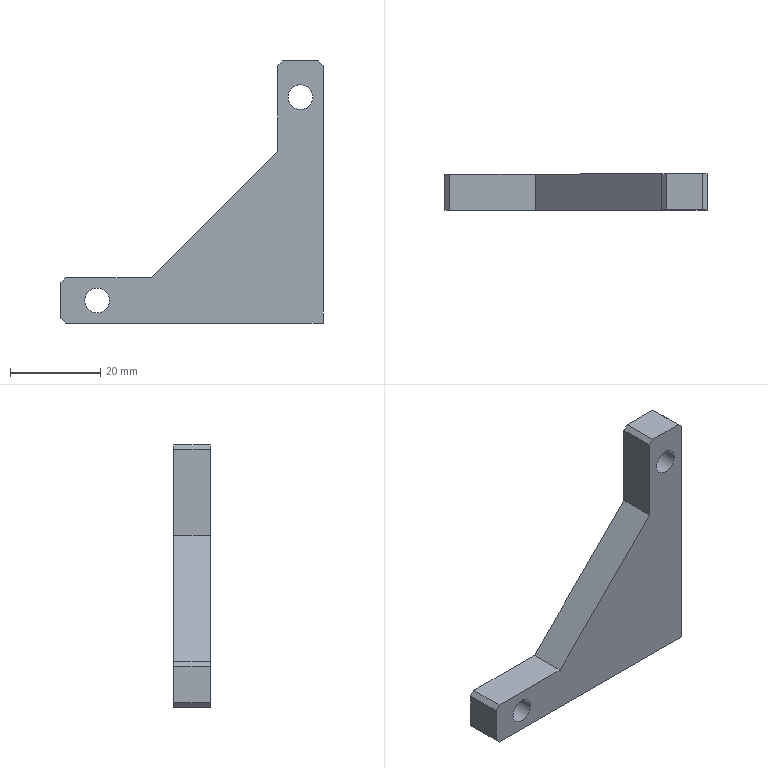Component | SolidWorks | MTCTV2104DJ006-000-0045RibPlate2-1 | 1 solid | 17 faces | box 58 x 8 x 58 mm | volume 11220 mm3 | plane 13 | cylinder 4 | commonest cylinder face diameters 5.5 x4
build123d program:
from build123d import *

# Parameters (mm, degrees)
SKETCH1_W                  = 8
SKETCH1_H                  = 58
BOSS_EXTRUDE1_DEPTH        = 58
CUT_EXTRUDE1_DEPTH         = 66.338
F_5_5_5_5_DIAMETER_HOLE1_D = 5.5
CHAMFER1_SIZE              = 1


with BuildPart() as part:
    # Sketch1 → Boss-Extrude1 (new body)
    with BuildSketch(Plane(origin=(0, 0, 0), x_dir=(0, 0, -1), z_dir=(1, 0, 0))):
        Rectangle(SKETCH1_W, SKETCH1_H)
    extrude(amount=BOSS_EXTRUDE1_DEPTH)

    # Sketch2 → Cut-Extrude1 (cut, through all)
    with BuildSketch(Plane.XY.offset(4)):
        Polygon((10, 29), (10, 9), (38, -19), (58, -19), (58, 29), align=None)
    extrude(amount=-CUT_EXTRUDE1_DEPTH, mode=Mode.SUBTRACT)

    # 5.5 _5.5_ Diameter Hole1 (through all)
    with Locations(Plane.XY.offset(4)):
        with Locations((5, 21), (50, -24)):
            Hole(F_5_5_5_5_DIAMETER_HOLE1_D / 2)

    # Chamfer1
    chamfer1_edges = [part.edges().sort_by_distance(p)[0] for p in [
        (58, -29, 0),
        (10, 29, 0),
        (58, -19, 0),
        (0, 29, 0),
    ]]
    chamfer(chamfer1_edges, length=CHAMFER1_SIZE)


solid = part.part

# Placed as in the assembly
solid = solid.moved(Location((30.798, 61.781, 171.447), (90, 0, 90)))
STEP:
#1=COLOUR_RGB('',0.7922,0.8196,0.9333);
#2=FILL_AREA_STYLE_COLOUR('',#1);
#3=FILL_AREA_STYLE('',(#2));
#4=SURFACE_STYLE_FILL_AREA(#3);
#5=SURFACE_SIDE_STYLE('',(#4));
#6=SURFACE_STYLE_USAGE(.BOTH.,#5);
#7=PRESENTATION_STYLE_ASSIGNMENT((#6));
#8=CARTESIAN_POINT('',(2.266,2.275,8.718));
#9=VERTEX_POINT('',#8);
#10=CARTESIAN_POINT('',(2.049,2.275,8.718));
#11=VERTEX_POINT('',#10);
#12=CARTESIAN_POINT('',(2.157,2.275,8.718));
#13=DIRECTION('',(-0.,1.,-0.));
#14=DIRECTION('',(-1.,0.,0.));
#15=AXIS2_PLACEMENT_3D('',#12,#13,#14);
#16=CIRCLE('',#15,0.1083);
#17=EDGE_CURVE('',#9,#11,#16,.T.);
#18=ORIENTED_EDGE('',*,*,#17,.F.);
#19=CARTESIAN_POINT('',(2.266,2.59,8.718));
#20=VERTEX_POINT('',#19);
#21=CARTESIAN_POINT('',(2.266,2.59,8.718));
#22=DIRECTION('',(-0.,1.,-0.));
#23=VECTOR('',#22,39.37);
#24=LINE('',#21,#23);
#25=EDGE_CURVE('',#9,#20,#24,.T.);
#26=ORIENTED_EDGE('',*,*,#25,.T.);
#27=CARTESIAN_POINT('',(2.049,2.59,8.718));
#28=VERTEX_POINT('',#27);
#29=CARTESIAN_POINT('',(2.157,2.59,8.718));
#30=DIRECTION('',(-0.,1.,-0.));
#31=DIRECTION('',(-1.,0.,0.));
#32=AXIS2_PLACEMENT_3D('',#29,#30,#31);
#33=CIRCLE('',#32,0.1083);
#34=EDGE_CURVE('',#20,#28,#33,.T.);
#35=ORIENTED_EDGE('',*,*,#34,.T.);
#36=CARTESIAN_POINT('',(2.049,2.59,8.718));
#37=DIRECTION('',(-0.,1.,-0.));
#38=VECTOR('',#37,39.37);
#39=LINE('',#36,#38);
#40=EDGE_CURVE('',#11,#28,#39,.T.);
#41=ORIENTED_EDGE('',*,*,#40,.F.);
#42=EDGE_LOOP('',(#18,#26,#35,#41));
#43=FACE_OUTER_BOUND('',#42,.T.);
#44=CARTESIAN_POINT('',(2.157,2.59,8.718));
#45=DIRECTION('',(-0.,1.,-0.));
#46=DIRECTION('',(-1.,0.,0.));
#47=AXIS2_PLACEMENT_3D('',#44,#45,#46);
#48=CYLINDRICAL_SURFACE('',#47,0.1083);
#49=ADVANCED_FACE('',(#43),#48,.F.);
#50=CARTESIAN_POINT('',(0.494,2.275,6.947));
#51=VERTEX_POINT('',#50);
#52=CARTESIAN_POINT('',(0.2775,2.275,6.947));
#53=VERTEX_POINT('',#52);
#54=CARTESIAN_POINT('',(0.3858,2.275,6.947));
#55=DIRECTION('',(-0.,1.,-0.));
#56=DIRECTION('',(-1.,0.,0.));
#57=AXIS2_PLACEMENT_3D('',#54,#55,#56);
#58=CIRCLE('',#57,0.1083);
#59=EDGE_CURVE('',#51,#53,#58,.T.);
#60=ORIENTED_EDGE('',*,*,#59,.F.);
#61=CARTESIAN_POINT('',(0.494,2.59,6.947));
#62=VERTEX_POINT('',#61);
#63=CARTESIAN_POINT('',(0.494,2.59,6.947));
#64=DIRECTION('',(-0.,1.,-0.));
#65=VECTOR('',#64,39.37);
#66=LINE('',#63,#65);
#67=EDGE_CURVE('',#51,#62,#66,.T.);
#68=ORIENTED_EDGE('',*,*,#67,.T.);
#69=CARTESIAN_POINT('',(0.2775,2.59,6.947));
#70=VERTEX_POINT('',#69);
#71=CARTESIAN_POINT('',(0.3858,2.59,6.947));
#72=DIRECTION('',(-0.,1.,-0.));
#73=DIRECTION('',(-1.,0.,0.));
#74=AXIS2_PLACEMENT_3D('',#71,#72,#73);
#75=CIRCLE('',#74,0.1083);
#76=EDGE_CURVE('',#62,#70,#75,.T.);
#77=ORIENTED_EDGE('',*,*,#76,.T.);
#78=CARTESIAN_POINT('',(0.2775,2.59,6.947));
#79=DIRECTION('',(-0.,1.,-0.));
#80=VECTOR('',#79,39.37);
#81=LINE('',#78,#80);
#82=EDGE_CURVE('',#53,#70,#81,.T.);
#83=ORIENTED_EDGE('',*,*,#82,.F.);
#84=EDGE_LOOP('',(#60,#68,#77,#83));
#85=FACE_OUTER_BOUND('',#84,.T.);
#86=CARTESIAN_POINT('',(0.3858,2.59,6.947));
#87=DIRECTION('',(-0.,1.,-0.));
#88=DIRECTION('',(-1.,0.,0.));
#89=AXIS2_PLACEMENT_3D('',#86,#87,#88);
#90=CYLINDRICAL_SURFACE('',#89,0.1083);
#91=ADVANCED_FACE('',(#85),#90,.F.);
#92=CARTESIAN_POINT('',(2.157,2.275,8.718));
#93=DIRECTION('',(-0.,1.,-0.));
#94=DIRECTION('',(-1.,0.,0.));
#95=AXIS2_PLACEMENT_3D('',#92,#93,#94);
#96=CIRCLE('',#95,0.1083);
#97=EDGE_CURVE('',#11,#9,#96,.T.);
#98=ORIENTED_EDGE('',*,*,#97,.T.);
#99=ORIENTED_EDGE('',*,*,#17,.T.);
#100=EDGE_LOOP('',(#98,#99));
#101=FACE_BOUND('',#100,.T.);
#102=CARTESIAN_POINT('',(0.3858,2.275,6.947));
#103=DIRECTION('',(-0.,1.,-0.));
#104=DIRECTION('',(-1.,0.,0.));
#105=AXIS2_PLACEMENT_3D('',#102,#103,#104);
#106=CIRCLE('',#105,0.1083);
#107=EDGE_CURVE('',#53,#51,#106,.T.);
#108=ORIENTED_EDGE('',*,*,#107,.T.);
#109=ORIENTED_EDGE('',*,*,#59,.T.);
#110=EDGE_LOOP('',(#108,#109));
#111=FACE_BOUND('',#110,.T.);
#112=CARTESIAN_POINT('',(0.07081,2.275,6.789));
#113=VERTEX_POINT('',#112);
#114=CARTESIAN_POINT('',(0.07081,2.275,7.104));
#115=VERTEX_POINT('',#114);
#116=CARTESIAN_POINT('',(0.07081,2.275,6.75));
#117=DIRECTION('',(-0.,0.,1.));
#118=VECTOR('',#117,39.37);
#119=LINE('',#116,#118);
#120=EDGE_CURVE('',#113,#115,#119,.T.);
#121=ORIENTED_EDGE('',*,*,#120,.F.);
#122=CARTESIAN_POINT('',(0.1102,2.275,6.75));
#123=VERTEX_POINT('',#122);
#124=CARTESIAN_POINT('',(0.07081,2.275,6.789));
#125=DIRECTION('',(0.7071,0.,-0.7071));
#126=VECTOR('',#125,39.37);
#127=LINE('',#124,#126);
#128=EDGE_CURVE('',#113,#123,#127,.T.);
#129=ORIENTED_EDGE('',*,*,#128,.T.);
#130=CARTESIAN_POINT('',(2.354,2.275,6.75));
#131=VERTEX_POINT('',#130);
#132=CARTESIAN_POINT('',(0.07081,2.275,6.75));
#133=DIRECTION('',(1.,0.,0.));
#134=VECTOR('',#133,39.37);
#135=LINE('',#132,#134);
#136=EDGE_CURVE('',#123,#131,#135,.T.);
#137=ORIENTED_EDGE('',*,*,#136,.T.);
#138=CARTESIAN_POINT('',(2.354,2.275,8.994));
#139=VERTEX_POINT('',#138);
#140=CARTESIAN_POINT('',(2.354,2.275,6.75));
#141=DIRECTION('',(-0.,0.,1.));
#142=VECTOR('',#141,39.37);
#143=LINE('',#140,#142);
#144=EDGE_CURVE('',#131,#139,#143,.T.);
#145=ORIENTED_EDGE('',*,*,#144,.T.);
#146=CARTESIAN_POINT('',(2.315,2.275,9.033));
#147=VERTEX_POINT('',#146);
#148=CARTESIAN_POINT('',(2.315,2.275,9.033));
#149=DIRECTION('',(-0.7071,-0.,0.7071));
#150=VECTOR('',#149,39.37);
#151=LINE('',#148,#150);
#152=EDGE_CURVE('',#139,#147,#151,.T.);
#153=ORIENTED_EDGE('',*,*,#152,.T.);
#154=CARTESIAN_POINT('',(2.,2.275,9.033));
#155=VERTEX_POINT('',#154);
#156=CARTESIAN_POINT('',(0.07081,2.275,9.033));
#157=DIRECTION('',(1.,0.,0.));
#158=VECTOR('',#157,39.37);
#159=LINE('',#156,#158);
#160=EDGE_CURVE('',#155,#147,#159,.T.);
#161=ORIENTED_EDGE('',*,*,#160,.F.);
#162=CARTESIAN_POINT('',(1.961,2.275,8.994));
#163=VERTEX_POINT('',#162);
#164=CARTESIAN_POINT('',(1.961,2.275,8.994));
#165=DIRECTION('',(-0.7071,-0.,-0.7071));
#166=VECTOR('',#165,39.37);
#167=LINE('',#164,#166);
#168=EDGE_CURVE('',#155,#163,#167,.T.);
#169=ORIENTED_EDGE('',*,*,#168,.T.);
#170=CARTESIAN_POINT('',(1.961,2.275,8.246));
#171=VERTEX_POINT('',#170);
#172=CARTESIAN_POINT('',(1.961,2.275,9.033));
#173=DIRECTION('',(0.,-0.,-1.));
#174=VECTOR('',#173,39.37);
#175=LINE('',#172,#174);
#176=EDGE_CURVE('',#163,#171,#175,.T.);
#177=ORIENTED_EDGE('',*,*,#176,.T.);
#178=CARTESIAN_POINT('',(0.8582,2.275,7.144));
#179=VERTEX_POINT('',#178);
#180=CARTESIAN_POINT('',(1.961,2.275,8.246));
#181=DIRECTION('',(-0.7071,-0.,-0.7071));
#182=VECTOR('',#181,39.37);
#183=LINE('',#180,#182);
#184=EDGE_CURVE('',#171,#179,#183,.T.);
#185=ORIENTED_EDGE('',*,*,#184,.T.);
#186=CARTESIAN_POINT('',(0.1102,2.275,7.144));
#187=VERTEX_POINT('',#186);
#188=CARTESIAN_POINT('',(0.8582,2.275,7.144));
#189=DIRECTION('',(-1.,-0.,-0.));
#190=VECTOR('',#189,39.37);
#191=LINE('',#188,#190);
#192=EDGE_CURVE('',#179,#187,#191,.T.);
#193=ORIENTED_EDGE('',*,*,#192,.T.);
#194=CARTESIAN_POINT('',(0.07081,2.275,7.104));
#195=DIRECTION('',(-0.7071,-0.,-0.7071));
#196=VECTOR('',#195,39.37);
#197=LINE('',#194,#196);
#198=EDGE_CURVE('',#187,#115,#197,.T.);
#199=ORIENTED_EDGE('',*,*,#198,.T.);
#200=EDGE_LOOP('',(#121,#129,#137,#145,#153,#161,#169,#177,#185,#193,#199));
#201=FACE_OUTER_BOUND('',#200,.T.);
#202=CARTESIAN_POINT('',(0.07081,2.275,6.75));
#203=DIRECTION('',(-0.,1.,-0.));
#204=DIRECTION('',(-1.,-0.,-0.));
#205=AXIS2_PLACEMENT_3D('',#202,#203,#204);
#206=PLANE('',#205);
#207=ADVANCED_FACE('',(#101,#111,#201),#206,.F.);
#208=ORIENTED_EDGE('',*,*,#160,.T.);
#209=CARTESIAN_POINT('',(2.315,2.59,9.033));
#210=VERTEX_POINT('',#209);
#211=CARTESIAN_POINT('',(2.315,2.59,9.033));
#212=DIRECTION('',(-0.,1.,-0.));
#213=VECTOR('',#212,39.37);
#214=LINE('',#211,#213);
#215=EDGE_CURVE('',#147,#210,#214,.T.);
#216=ORIENTED_EDGE('',*,*,#215,.T.);
#217=CARTESIAN_POINT('',(2.,2.59,9.033));
#218=VERTEX_POINT('',#217);
#219=CARTESIAN_POINT('',(0.07081,2.59,9.033));
#220=DIRECTION('',(1.,0.,0.));
#221=VECTOR('',#220,39.37);
#222=LINE('',#219,#221);
#223=EDGE_CURVE('',#218,#210,#222,.T.);
#224=ORIENTED_EDGE('',*,*,#223,.F.);
#225=CARTESIAN_POINT('',(2.,2.59,9.033));
#226=DIRECTION('',(0.,-1.,0.));
#227=VECTOR('',#226,39.37);
#228=LINE('',#225,#227);
#229=EDGE_CURVE('',#218,#155,#228,.T.);
#230=ORIENTED_EDGE('',*,*,#229,.T.);
#231=EDGE_LOOP('',(#208,#216,#224,#230));
#232=FACE_OUTER_BOUND('',#231,.T.);
#233=CARTESIAN_POINT('',(0.07081,2.59,9.033));
#234=DIRECTION('',(0.,-0.,-1.));
#235=DIRECTION('',(0.,-1.,0.));
#236=AXIS2_PLACEMENT_3D('',#233,#234,#235);
#237=PLANE('',#236);
#238=ADVANCED_FACE('',(#232),#237,.F.);
#239=CARTESIAN_POINT('',(2.157,2.59,8.718));
#240=DIRECTION('',(-0.,1.,-0.));
#241=DIRECTION('',(-1.,0.,0.));
#242=AXIS2_PLACEMENT_3D('',#239,#240,#241);
#243=CIRCLE('',#242,0.1083);
#244=EDGE_CURVE('',#28,#20,#243,.T.);
#245=ORIENTED_EDGE('',*,*,#244,.F.);
#246=ORIENTED_EDGE('',*,*,#34,.F.);
#247=EDGE_LOOP('',(#245,#246));
#248=FACE_BOUND('',#247,.T.);
#249=CARTESIAN_POINT('',(0.3858,2.59,6.947));
#250=DIRECTION('',(-0.,1.,-0.));
#251=DIRECTION('',(-1.,0.,0.));
#252=AXIS2_PLACEMENT_3D('',#249,#250,#251);
#253=CIRCLE('',#252,0.1083);
#254=EDGE_CURVE('',#70,#62,#253,.T.);
#255=ORIENTED_EDGE('',*,*,#254,.F.);
#256=ORIENTED_EDGE('',*,*,#76,.F.);
#257=EDGE_LOOP('',(#255,#256));
#258=FACE_BOUND('',#257,.T.);
#259=CARTESIAN_POINT('',(0.1102,2.59,6.75));
#260=VERTEX_POINT('',#259);
#261=CARTESIAN_POINT('',(2.354,2.59,6.75));
#262=VERTEX_POINT('',#261);
#263=CARTESIAN_POINT('',(0.07081,2.59,6.75));
#264=DIRECTION('',(1.,0.,0.));
#265=VECTOR('',#264,39.37);
#266=LINE('',#263,#265);
#267=EDGE_CURVE('',#260,#262,#266,.T.);
#268=ORIENTED_EDGE('',*,*,#267,.F.);
#269=CARTESIAN_POINT('',(0.07081,2.59,6.789));
#270=VERTEX_POINT('',#269);
#271=CARTESIAN_POINT('',(0.07081,2.59,6.789));
#272=DIRECTION('',(-0.7071,-0.,0.7071));
#273=VECTOR('',#272,39.37);
#274=LINE('',#271,#273);
#275=EDGE_CURVE('',#260,#270,#274,.T.);
#276=ORIENTED_EDGE('',*,*,#275,.T.);
#277=CARTESIAN_POINT('',(0.07081,2.59,7.104));
#278=VERTEX_POINT('',#277);
#279=CARTESIAN_POINT('',(0.07081,2.59,6.75));
#280=DIRECTION('',(0.,-0.,-1.));
#281=VECTOR('',#280,39.37);
#282=LINE('',#279,#281);
#283=EDGE_CURVE('',#278,#270,#282,.T.);
#284=ORIENTED_EDGE('',*,*,#283,.F.);
#285=CARTESIAN_POINT('',(0.1102,2.59,7.144));
#286=VERTEX_POINT('',#285);
#287=CARTESIAN_POINT('',(0.07081,2.59,7.104));
#288=DIRECTION('',(0.7071,0.,0.7071));
#289=VECTOR('',#288,39.37);
#290=LINE('',#287,#289);
#291=EDGE_CURVE('',#278,#286,#290,.T.);
#292=ORIENTED_EDGE('',*,*,#291,.T.);
#293=CARTESIAN_POINT('',(0.8582,2.59,7.144));
#294=VERTEX_POINT('',#293);
#295=CARTESIAN_POINT('',(0.8582,2.59,7.144));
#296=DIRECTION('',(-1.,-0.,-0.));
#297=VECTOR('',#296,39.37);
#298=LINE('',#295,#297);
#299=EDGE_CURVE('',#294,#286,#298,.T.);
#300=ORIENTED_EDGE('',*,*,#299,.F.);
#301=CARTESIAN_POINT('',(1.961,2.59,8.246));
#302=VERTEX_POINT('',#301);
#303=CARTESIAN_POINT('',(1.961,2.59,8.246));
#304=DIRECTION('',(-0.7071,-0.,-0.7071));
#305=VECTOR('',#304,39.37);
#306=LINE('',#303,#305);
#307=EDGE_CURVE('',#302,#294,#306,.T.);
#308=ORIENTED_EDGE('',*,*,#307,.F.);
#309=CARTESIAN_POINT('',(1.961,2.59,8.994));
#310=VERTEX_POINT('',#309);
#311=CARTESIAN_POINT('',(1.961,2.59,9.033));
#312=DIRECTION('',(0.,-0.,-1.));
#313=VECTOR('',#312,39.37);
#314=LINE('',#311,#313);
#315=EDGE_CURVE('',#310,#302,#314,.T.);
#316=ORIENTED_EDGE('',*,*,#315,.F.);
#317=CARTESIAN_POINT('',(1.961,2.59,8.994));
#318=DIRECTION('',(0.7071,0.,0.7071));
#319=VECTOR('',#318,39.37);
#320=LINE('',#317,#319);
#321=EDGE_CURVE('',#310,#218,#320,.T.);
#322=ORIENTED_EDGE('',*,*,#321,.T.);
#323=ORIENTED_EDGE('',*,*,#223,.T.);
#324=CARTESIAN_POINT('',(2.354,2.59,8.994));
#325=VERTEX_POINT('',#324);
#326=CARTESIAN_POINT('',(2.315,2.59,9.033));
#327=DIRECTION('',(0.7071,0.,-0.7071));
#328=VECTOR('',#327,39.37);
#329=LINE('',#326,#328);
#330=EDGE_CURVE('',#210,#325,#329,.T.);
#331=ORIENTED_EDGE('',*,*,#330,.T.);
#332=CARTESIAN_POINT('',(2.354,2.59,6.75));
#333=DIRECTION('',(0.,-0.,-1.));
#334=VECTOR('',#333,39.37);
#335=LINE('',#332,#334);
#336=EDGE_CURVE('',#325,#262,#335,.T.);
#337=ORIENTED_EDGE('',*,*,#336,.T.);
#338=EDGE_LOOP('',(#268,#276,#284,#292,#300,#308,#316,#322,#323,#331,#337));
#339=FACE_OUTER_BOUND('',#338,.T.);
#340=CARTESIAN_POINT('',(0.07081,2.59,6.75));
#341=DIRECTION('',(0.,-1.,0.));
#342=DIRECTION('',(1.,0.,0.));
#343=AXIS2_PLACEMENT_3D('',#340,#341,#342);
#344=PLANE('',#343);
#345=ADVANCED_FACE('',(#248,#258,#339),#344,.F.);
#346=ORIENTED_EDGE('',*,*,#136,.F.);
#347=CARTESIAN_POINT('',(0.1102,2.59,6.75));
#348=DIRECTION('',(-0.,1.,-0.));
#349=VECTOR('',#348,39.37);
#350=LINE('',#347,#349);
#351=EDGE_CURVE('',#123,#260,#350,.T.);
#352=ORIENTED_EDGE('',*,*,#351,.T.);
#353=ORIENTED_EDGE('',*,*,#267,.T.);
#354=CARTESIAN_POINT('',(2.354,2.59,6.75));
#355=DIRECTION('',(0.,-1.,0.));
#356=VECTOR('',#355,39.37);
#357=LINE('',#354,#356);
#358=EDGE_CURVE('',#262,#131,#357,.T.);
#359=ORIENTED_EDGE('',*,*,#358,.T.);
#360=EDGE_LOOP('',(#346,#352,#353,#359));
#361=FACE_OUTER_BOUND('',#360,.T.);
#362=CARTESIAN_POINT('',(0.07081,2.59,6.75));
#363=DIRECTION('',(-0.,0.,1.));
#364=DIRECTION('',(-0.,1.,-0.));
#365=AXIS2_PLACEMENT_3D('',#362,#363,#364);
#366=PLANE('',#365);
#367=ADVANCED_FACE('',(#361),#366,.F.);
#368=ORIENTED_EDGE('',*,*,#283,.T.);
#369=CARTESIAN_POINT('',(0.07081,2.432,6.789));
#370=DIRECTION('',(0.,-1.,0.));
#371=VECTOR('',#370,39.37);
#372=LINE('',#369,#371);
#373=EDGE_CURVE('',#270,#113,#372,.T.);
#374=ORIENTED_EDGE('',*,*,#373,.T.);
#375=ORIENTED_EDGE('',*,*,#120,.T.);
#376=CARTESIAN_POINT('',(0.07081,2.432,7.104));
#377=DIRECTION('',(-0.,1.,-0.));
#378=VECTOR('',#377,39.37);
#379=LINE('',#376,#378);
#380=EDGE_CURVE('',#115,#278,#379,.T.);
#381=ORIENTED_EDGE('',*,*,#380,.T.);
#382=EDGE_LOOP('',(#368,#374,#375,#381));
#383=FACE_OUTER_BOUND('',#382,.T.);
#384=CARTESIAN_POINT('',(0.07081,2.432,7.892));
#385=DIRECTION('',(1.,0.,0.));
#386=DIRECTION('',(-0.,1.,-0.));
#387=AXIS2_PLACEMENT_3D('',#384,#385,#386);
#388=PLANE('',#387);
#389=ADVANCED_FACE('',(#383),#388,.F.);
#390=ORIENTED_EDGE('',*,*,#336,.F.);
#391=CARTESIAN_POINT('',(2.354,2.275,8.994));
#392=DIRECTION('',(0.,-1.,0.));
#393=VECTOR('',#392,39.37);
#394=LINE('',#391,#393);
#395=EDGE_CURVE('',#325,#139,#394,.T.);
#396=ORIENTED_EDGE('',*,*,#395,.T.);
#397=ORIENTED_EDGE('',*,*,#144,.F.);
#398=ORIENTED_EDGE('',*,*,#358,.F.);
#399=EDGE_LOOP('',(#390,#396,#397,#398));
#400=FACE_OUTER_BOUND('',#399,.T.);
#401=CARTESIAN_POINT('',(2.354,2.432,7.892));
#402=DIRECTION('',(1.,0.,0.));
#403=DIRECTION('',(-0.,1.,-0.));
#404=AXIS2_PLACEMENT_3D('',#401,#402,#403);
#405=PLANE('',#404);
#406=ADVANCED_FACE('',(#400),#405,.T.);
#407=ORIENTED_EDGE('',*,*,#299,.T.);
#408=CARTESIAN_POINT('',(0.1102,2.275,7.144));
#409=DIRECTION('',(0.,-1.,0.));
#410=VECTOR('',#409,39.37);
#411=LINE('',#408,#410);
#412=EDGE_CURVE('',#286,#187,#411,.T.);
#413=ORIENTED_EDGE('',*,*,#412,.T.);
#414=ORIENTED_EDGE('',*,*,#192,.F.);
#415=CARTESIAN_POINT('',(0.8582,2.275,7.144));
#416=DIRECTION('',(-0.,1.,-0.));
#417=VECTOR('',#416,39.37);
#418=LINE('',#415,#417);
#419=EDGE_CURVE('',#179,#294,#418,.T.);
#420=ORIENTED_EDGE('',*,*,#419,.T.);
#421=EDGE_LOOP('',(#407,#413,#414,#420));
#422=FACE_OUTER_BOUND('',#421,.T.);
#423=CARTESIAN_POINT('',(0.8582,2.275,7.144));
#424=DIRECTION('',(0.,-0.,-1.));
#425=DIRECTION('',(0.,-1.,0.));
#426=AXIS2_PLACEMENT_3D('',#423,#424,#425);
#427=PLANE('',#426);
#428=ADVANCED_FACE('',(#422),#427,.F.);
#429=ORIENTED_EDGE('',*,*,#307,.T.);
#430=ORIENTED_EDGE('',*,*,#419,.F.);
#431=ORIENTED_EDGE('',*,*,#184,.F.);
#432=CARTESIAN_POINT('',(1.961,2.275,8.246));
#433=DIRECTION('',(-0.,1.,-0.));
#434=VECTOR('',#433,39.37);
#435=LINE('',#432,#434);
#436=EDGE_CURVE('',#171,#302,#435,.T.);
#437=ORIENTED_EDGE('',*,*,#436,.T.);
#438=EDGE_LOOP('',(#429,#430,#431,#437));
#439=FACE_OUTER_BOUND('',#438,.T.);
#440=CARTESIAN_POINT('',(1.961,2.275,8.246));
#441=DIRECTION('',(0.7071,0.,-0.7071));
#442=DIRECTION('',(-0.7071,-0.,-0.7071));
#443=AXIS2_PLACEMENT_3D('',#440,#441,#442);
#444=PLANE('',#443);
#445=ADVANCED_FACE('',(#439),#444,.F.);
#446=ORIENTED_EDGE('',*,*,#176,.F.);
#447=CARTESIAN_POINT('',(1.961,2.275,8.994));
#448=DIRECTION('',(-0.,1.,-0.));
#449=VECTOR('',#448,39.37);
#450=LINE('',#447,#449);
#451=EDGE_CURVE('',#163,#310,#450,.T.);
#452=ORIENTED_EDGE('',*,*,#451,.T.);
#453=ORIENTED_EDGE('',*,*,#315,.T.);
#454=ORIENTED_EDGE('',*,*,#436,.F.);
#455=EDGE_LOOP('',(#446,#452,#453,#454));
#456=FACE_OUTER_BOUND('',#455,.T.);
#457=CARTESIAN_POINT('',(1.961,2.275,9.033));
#458=DIRECTION('',(1.,0.,0.));
#459=DIRECTION('',(0.,-0.,-1.));
#460=AXIS2_PLACEMENT_3D('',#457,#458,#459);
#461=PLANE('',#460);
#462=ADVANCED_FACE('',(#456),#461,.F.);
#463=ORIENTED_EDGE('',*,*,#67,.F.);
#464=ORIENTED_EDGE('',*,*,#107,.F.);
#465=ORIENTED_EDGE('',*,*,#82,.T.);
#466=ORIENTED_EDGE('',*,*,#254,.T.);
#467=EDGE_LOOP('',(#463,#464,#465,#466));
#468=FACE_OUTER_BOUND('',#467,.T.);
#469=CARTESIAN_POINT('',(0.3858,2.59,6.947));
#470=DIRECTION('',(-0.,1.,-0.));
#471=DIRECTION('',(-1.,0.,0.));
#472=AXIS2_PLACEMENT_3D('',#469,#470,#471);
#473=CYLINDRICAL_SURFACE('',#472,0.1083);
#474=ADVANCED_FACE('',(#468),#473,.F.);
#475=ORIENTED_EDGE('',*,*,#25,.F.);
#476=ORIENTED_EDGE('',*,*,#97,.F.);
#477=ORIENTED_EDGE('',*,*,#40,.T.);
#478=ORIENTED_EDGE('',*,*,#244,.T.);
#479=EDGE_LOOP('',(#475,#476,#477,#478));
#480=FACE_OUTER_BOUND('',#479,.T.);
#481=CARTESIAN_POINT('',(2.157,2.59,8.718));
#482=DIRECTION('',(-0.,1.,-0.));
#483=DIRECTION('',(-1.,0.,0.));
#484=AXIS2_PLACEMENT_3D('',#481,#482,#483);
#485=CYLINDRICAL_SURFACE('',#484,0.1083);
#486=ADVANCED_FACE('',(#480),#485,.F.);
#487=ORIENTED_EDGE('',*,*,#275,.F.);
#488=ORIENTED_EDGE('',*,*,#351,.F.);
#489=ORIENTED_EDGE('',*,*,#128,.F.);
#490=ORIENTED_EDGE('',*,*,#373,.F.);
#491=EDGE_LOOP('',(#487,#488,#489,#490));
#492=FACE_OUTER_BOUND('',#491,.T.);
#493=CARTESIAN_POINT('',(0.07081,2.432,6.789));
#494=DIRECTION('',(0.7071,0.,0.7071));
#495=DIRECTION('',(0.,-1.,0.));
#496=AXIS2_PLACEMENT_3D('',#493,#494,#495);
#497=PLANE('',#496);
#498=ADVANCED_FACE('',(#492),#497,.F.);
#499=ORIENTED_EDGE('',*,*,#198,.F.);
#500=ORIENTED_EDGE('',*,*,#412,.F.);
#501=ORIENTED_EDGE('',*,*,#291,.F.);
#502=ORIENTED_EDGE('',*,*,#380,.F.);
#503=EDGE_LOOP('',(#499,#500,#501,#502));
#504=FACE_OUTER_BOUND('',#503,.T.);
#505=CARTESIAN_POINT('',(0.07081,2.432,7.104));
#506=DIRECTION('',(0.7071,0.,-0.7071));
#507=DIRECTION('',(-0.,1.,-0.));
#508=AXIS2_PLACEMENT_3D('',#505,#506,#507);
#509=PLANE('',#508);
#510=ADVANCED_FACE('',(#504),#509,.F.);
#511=ORIENTED_EDGE('',*,*,#152,.F.);
#512=ORIENTED_EDGE('',*,*,#395,.F.);
#513=ORIENTED_EDGE('',*,*,#330,.F.);
#514=ORIENTED_EDGE('',*,*,#215,.F.);
#515=EDGE_LOOP('',(#511,#512,#513,#514));
#516=FACE_OUTER_BOUND('',#515,.T.);
#517=CARTESIAN_POINT('',(2.315,2.59,9.033));
#518=DIRECTION('',(0.7071,0.,0.7071));
#519=DIRECTION('',(0.,-1.,0.));
#520=AXIS2_PLACEMENT_3D('',#517,#518,#519);
#521=PLANE('',#520);
#522=ADVANCED_FACE('',(#516),#521,.T.);
#523=ORIENTED_EDGE('',*,*,#168,.F.);
#524=ORIENTED_EDGE('',*,*,#229,.F.);
#525=ORIENTED_EDGE('',*,*,#321,.F.);
#526=ORIENTED_EDGE('',*,*,#451,.F.);
#527=EDGE_LOOP('',(#523,#524,#525,#526));
#528=FACE_OUTER_BOUND('',#527,.T.);
#529=CARTESIAN_POINT('',(1.961,2.275,8.994));
#530=DIRECTION('',(0.7071,0.,-0.7071));
#531=DIRECTION('',(-0.,1.,-0.));
#532=AXIS2_PLACEMENT_3D('',#529,#530,#531);
#533=PLANE('',#532);
#534=ADVANCED_FACE('',(#528),#533,.F.);
#535=CLOSED_SHELL('',(#49,#91,#207,#238,#345,#367,#389,#406,#428,#445,#462,#474,#486,#498,#510,#522,#534));
#536=MANIFOLD_SOLID_BREP('',#535);
#537=STYLED_ITEM('',(#7),#536);
#538=PRESENTATION_LAYER_ASSIGNMENT('','',(#537));
#539=CARTESIAN_POINT('',(0.,0.,0.));
#540=DIRECTION('',(0.,0.,1.));
#541=DIRECTION('',(1.,0.,0.));
#542=AXIS2_PLACEMENT_3D('',#539,#540,#541);
#543=(LENGTH_UNIT()NAMED_UNIT(*)SI_UNIT($,.METRE.));
#544=LENGTH_MEASURE_WITH_UNIT(LENGTH_MEASURE(0.0254),#543);
#545=DIMENSIONAL_EXPONENTS(1.,0.,0.,0.,0.,0.,0.);
#546=(CONVERSION_BASED_UNIT('',#544)LENGTH_UNIT()NAMED_UNIT(#545));
#547=UNCERTAINTY_MEASURE_WITH_UNIT(LENGTH_MEASURE(0.00001),#546,'','');
#548=(NAMED_UNIT(*)PLANE_ANGLE_UNIT()SI_UNIT($,.RADIAN.));
#549=(NAMED_UNIT(*)SI_UNIT($,.STERADIAN.)SOLID_ANGLE_UNIT());
#550=(GEOMETRIC_REPRESENTATION_CONTEXT(3)GLOBAL_UNCERTAINTY_ASSIGNED_CONTEXT((#547))GLOBAL_UNIT_ASSIGNED_CONTEXT((#546,#548,#549))REPRESENTATION_CONTEXT('',''));
#551=ADVANCED_BREP_SHAPE_REPRESENTATION('',(#536,#542),#550);
#552=(LENGTH_UNIT()NAMED_UNIT(*)SI_UNIT($,.METRE.));
#553=LENGTH_MEASURE_WITH_UNIT(LENGTH_MEASURE(0.0254),#552);
#554=DIMENSIONAL_EXPONENTS(1.,0.,0.,0.,0.,0.,0.);
#555=(CONVERSION_BASED_UNIT('',#553)LENGTH_UNIT()NAMED_UNIT(#554));
#556=UNCERTAINTY_MEASURE_WITH_UNIT(LENGTH_MEASURE(0.00001),#555,'','');
#557=(NAMED_UNIT(*)PLANE_ANGLE_UNIT()SI_UNIT($,.RADIAN.));
#558=(NAMED_UNIT(*)SI_UNIT($,.STERADIAN.)SOLID_ANGLE_UNIT());
#559=(GEOMETRIC_REPRESENTATION_CONTEXT(3)GLOBAL_UNCERTAINTY_ASSIGNED_CONTEXT((#556))GLOBAL_UNIT_ASSIGNED_CONTEXT((#555,#557,#558))REPRESENTATION_CONTEXT('',''));
#560=MECHANICAL_DESIGN_GEOMETRIC_PRESENTATION_REPRESENTATION('',(#537),#559);